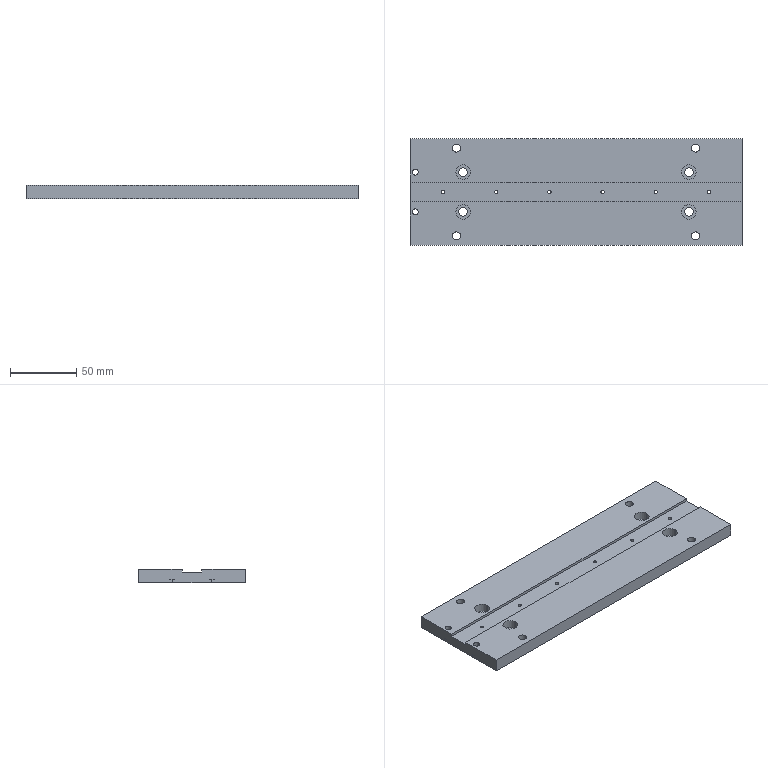CAM job | Mastercam | mm | 4 operations | part box 250 x 80 x 10
1. Contour (Ramp) | 1 - 8C
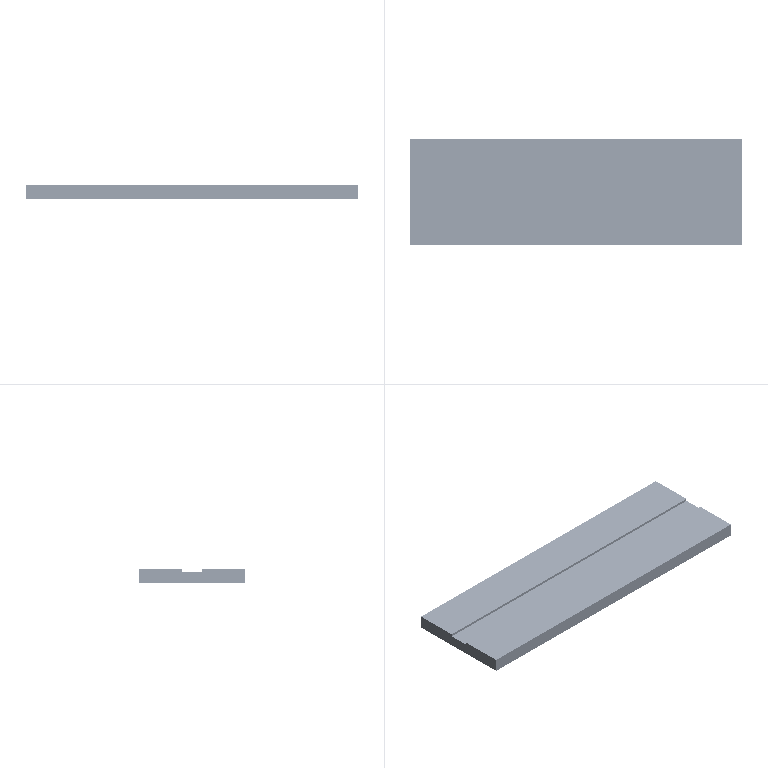2. Contour (2D) | 2 - 8J
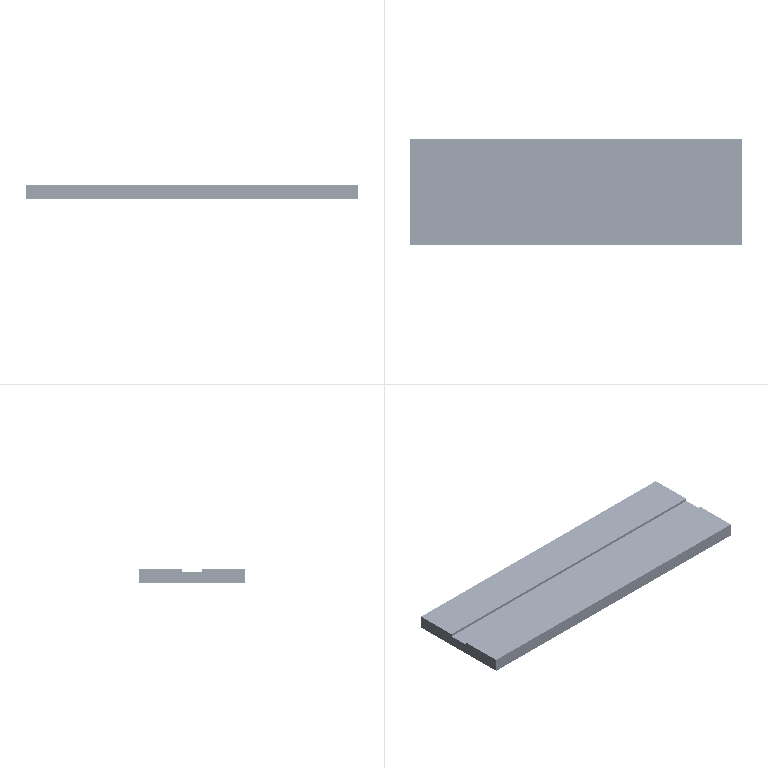3. Model Chamfer | 3 - 6 倒角刀
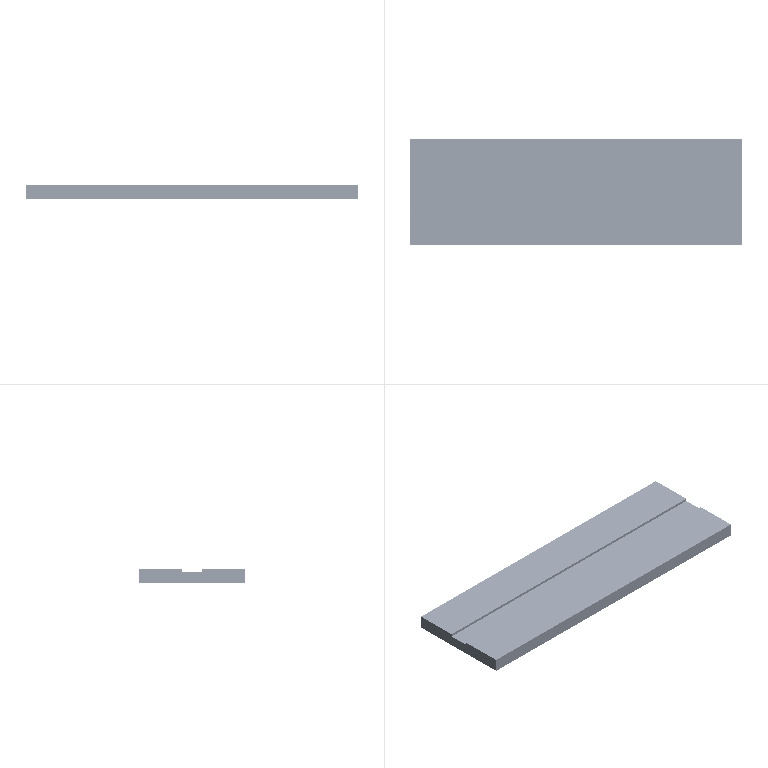4. Drill/Counterbore | 3 - 6 倒角刀